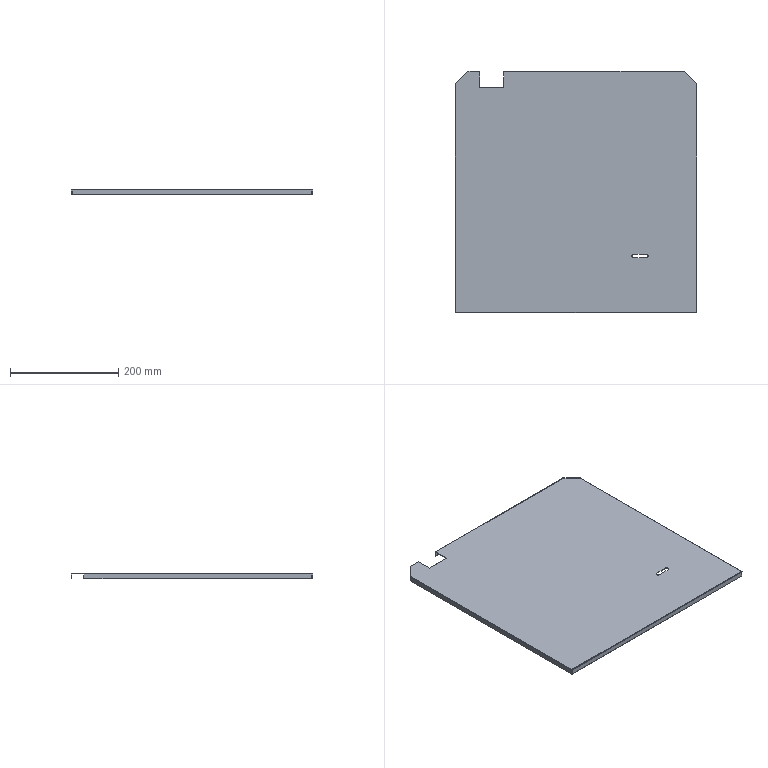Component | SolidWorks | WeldmentDrawing-1_Partition-1 | 1 solid | 61 faces | volume 212060 mm3 | plane 44 | cylinder 13 | spline 4 | commonest cylinder face diameters 2.2 x5 0.2 x5 7 x3